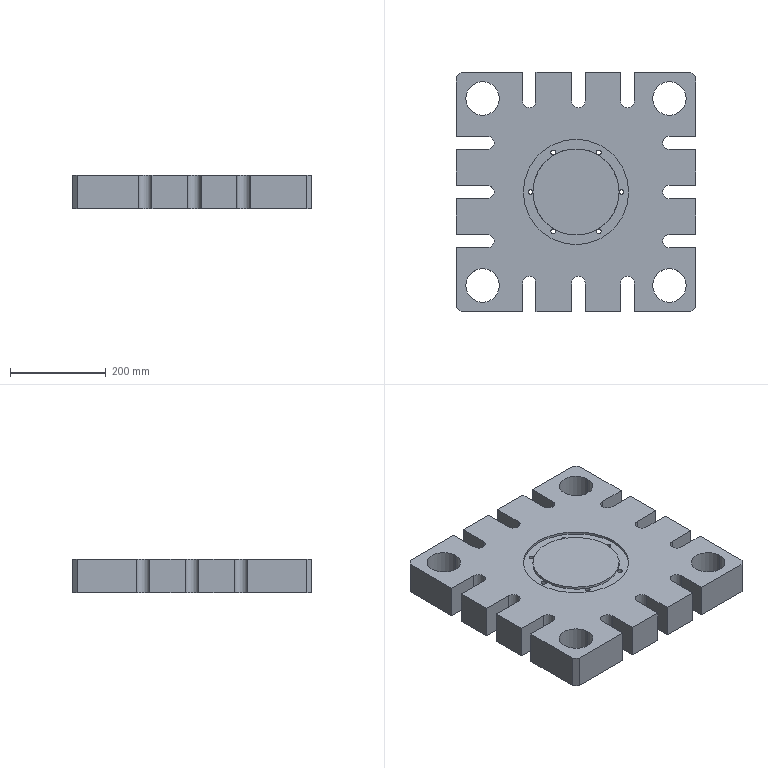Component | SolidWorks | UpperDiePlate-1 | 1 solid | 117 faces | box 500 x 500 x 70 mm | volume 14515565 mm3 | cylinder 59 | plane 58 | commonest cylinder face diameters 28 x15 20 x12 10 x12 80 x8 70 x8 180 x2 220 x2
build123d program:
from build123d import *

# Parameters (mm, degrees)
SKETCH2_W                 = 500
SKETCH2_H                 = 500
BOSS_EXTRUDE1_DEPTH       = 70
SKETCH3_R                 = 35
CUT_EXTRUDE1_DEPTH        = 361.416
CUT_EXTRUDE2_DEPTH        = 361.416
CHAMFER1_SIZE             = 10
SKETCH5_R                 = 40
CUT_EXTRUDE3_DEPTH        = 20
SKETCH6_R                 = 110
SKETCH6_R_2               = 90
CUT_EXTRUDE4_DEPTH        = 5
SIZE_MM_DOWEL_PIN_HOLE1_D = 10
SKETCH9_R                 = 10
CUT_EXTRUDE5_DEPTH        = 25


with BuildPart() as part:
    # Sketch2 → Boss-Extrude1 (new body)
    with BuildSketch(Plane.XY):
        Rectangle(SKETCH2_W, SKETCH2_H)
    extrude(amount=BOSS_EXTRUDE1_DEPTH)

    # Sketch3 → Cut-Extrude1 (cut, through all)
    with BuildSketch(Plane.XY.offset(70)):
        with Locations((-195, 195)):
            Circle(SKETCH3_R)
        with Locations(Location((195, 195, 0), (0, 0, 180))):
            Circle(SKETCH3_R)
        with Locations((195, -195)):
            Circle(SKETCH3_R)
        with Locations(Location((-195, -195, 0), (0, 0, 180))):
            Circle(SKETCH3_R)
    extrude(amount=-CUT_EXTRUDE1_DEPTH, mode=Mode.SUBTRACT)

    # Sketch4 → Cut-Extrude2 (cut, through all)
    with BuildSketch(Plane.XY.offset(70)):
        with BuildLine():
            Line((-195, 14), (-276.463, 14))
            Line((-276.463, 14), (-276.463, -14))
            Line((-276.463, -14), (-195, -14))
            ThreePointArc((-195, -14), (-181, 0), (-195, 14))
        make_face()
        with BuildLine():
            Line((-195, -88.5), (-276.463, -88.5))
            Line((-276.463, -88.5), (-276.463, -116.5))
            Line((-276.463, -116.5), (-195, -116.5))
            ThreePointArc((-195, -116.5), (-181, -102.5), (-195, -88.5))
        make_face()
        with BuildLine():
            Line((-276.463, 116.5), (-195, 116.5))
            ThreePointArc((-195, 116.5), (-181, 102.5), (-195, 88.5))
            Line((-195, 88.5), (-276.463, 88.5))
            Line((-276.463, 88.5), (-276.463, 116.5))
        make_face()
        with BuildLine():
            Line((83.5, 190), (83.5, 271.463))
            Line((83.5, 271.463), (111.5, 271.463))
            Line((111.5, 271.463), (111.5, 190))
            ThreePointArc((111.5, 190), (97.5, 176), (83.5, 190))
        make_face()
        with BuildLine():
            Line((9, 190), (9, 271.463))
            Line((9, 271.463), (-19, 271.463))
            Line((-19, 271.463), (-19, 190))
            ThreePointArc((-19, 190), (-5, 176), (9, 190))
        make_face()
        with BuildLine():
            Line((-93.5, 190), (-93.5, 271.463))
            Line((-93.5, 271.463), (-121.5, 271.463))
            Line((-121.5, 271.463), (-121.5, 190))
            ThreePointArc((-121.5, 190), (-107.5, 176), (-93.5, 190))
        make_face()
        with BuildLine():
            Line((185, -88.5), (266.463, -88.5))
            Line((266.463, -88.5), (266.463, -116.5))
            Line((266.463, -116.5), (185, -116.5))
            ThreePointArc((185, -116.5), (171, -102.5), (185, -88.5))
        make_face()
        with BuildLine():
            Line((185, -14), (266.463, -14))
            Line((266.463, -14), (266.463, 14))
            Line((266.463, 14), (185, 14))
            ThreePointArc((185, 14), (171, 0), (185, -14))
        make_face()
        with BuildLine():
            Line((185, 88.5), (266.463, 88.5))
            Line((266.463, 88.5), (266.463, 116.5))
            Line((266.463, 116.5), (185, 116.5))
            ThreePointArc((185, 116.5), (171, 102.5), (185, 88.5))
        make_face()
        with BuildLine():
            Line((-93.5, -190), (-93.5, -271.463))
            Line((-93.5, -271.463), (-121.5, -271.463))
            Line((-121.5, -271.463), (-121.5, -190))
            ThreePointArc((-121.5, -190), (-107.5, -176), (-93.5, -190))
        make_face()
        with BuildLine():
            Line((-19, -190), (-19, -271.463))
            Line((-19, -271.463), (9, -271.463))
            Line((9, -271.463), (9, -190))
            ThreePointArc((9, -190), (-5, -176), (-19, -190))
        make_face()
        with BuildLine():
            Line((83.5, -190), (83.5, -271.463))
            Line((83.5, -271.463), (111.5, -271.463))
            Line((111.5, -271.463), (111.5, -190))
            ThreePointArc((111.5, -190), (97.5, -176), (83.5, -190))
        make_face()
    extrude(amount=-CUT_EXTRUDE2_DEPTH, mode=Mode.SUBTRACT)

    # Chamfer1
    chamfer1_edges = [part.edges().sort_by_distance(p)[0] for p in [
        (250, -250, 35),
        (-250, -250, 35),
        (-250, 250, 35),
        (250, 250, 35),
    ]]
    chamfer(chamfer1_edges, length=CHAMFER1_SIZE)

    # Sketch5 → Cut-Extrude3 (cut)
    with BuildSketch(Plane.XY.offset(70)):
        with Locations((-195, 195)):
            Circle(SKETCH5_R)
        with Locations((195, 195)):
            Circle(SKETCH5_R)
        with Locations((195, -195)):
            Circle(SKETCH5_R)
        with Locations((-195, -195)):
            Circle(SKETCH5_R)
    extrude(amount=-CUT_EXTRUDE3_DEPTH, mode=Mode.SUBTRACT)

    # Sketch6 → Cut-Extrude4 (cut)
    with BuildSketch(Plane(origin=(0, 0, 0), x_dir=(-1, 0, 0), z_dir=(0, 0, -1))):
        Circle(SKETCH6_R)
        Circle(SKETCH6_R_2, mode=Mode.SUBTRACT)
    extrude(amount=-CUT_EXTRUDE4_DEPTH, mode=Mode.SUBTRACT)

    # Size mm Dowel Pin Hole1 (through all)
    with Locations(Plane(origin=(0, 0, 5), x_dir=(-1, 0, 0), z_dir=(0, 0, -1))):
        with Locations((-47.5, 82.272), (-95, 0), (-47.5, -82.272), (47.5, -82.272), (95, 0), (47.5, 82.272)):
            Hole(SIZE_MM_DOWEL_PIN_HOLE1_D / 2)

    # Sketch9 → Cut-Extrude5 (cut)
    with BuildSketch(Plane.XY.offset(70)):
        with Locations((-95, 0)):
            Circle(SKETCH9_R)
        with Locations((-47.5, 82.272)):
            Circle(SKETCH9_R)
        with Locations((47.5, 82.272)):
            Circle(SKETCH9_R)
        with Locations((95, 0)):
            Circle(SKETCH9_R)
        with Locations((47.5, -82.272)):
            Circle(SKETCH9_R)
        with Locations((-47.5, -82.272)):
            Circle(SKETCH9_R)
    extrude(amount=-CUT_EXTRUDE5_DEPTH, mode=Mode.SUBTRACT)


solid = part.part

# Placed as in the assembly
solid = solid.moved(Location((0, 0, -271), (-180, 0, 180)))